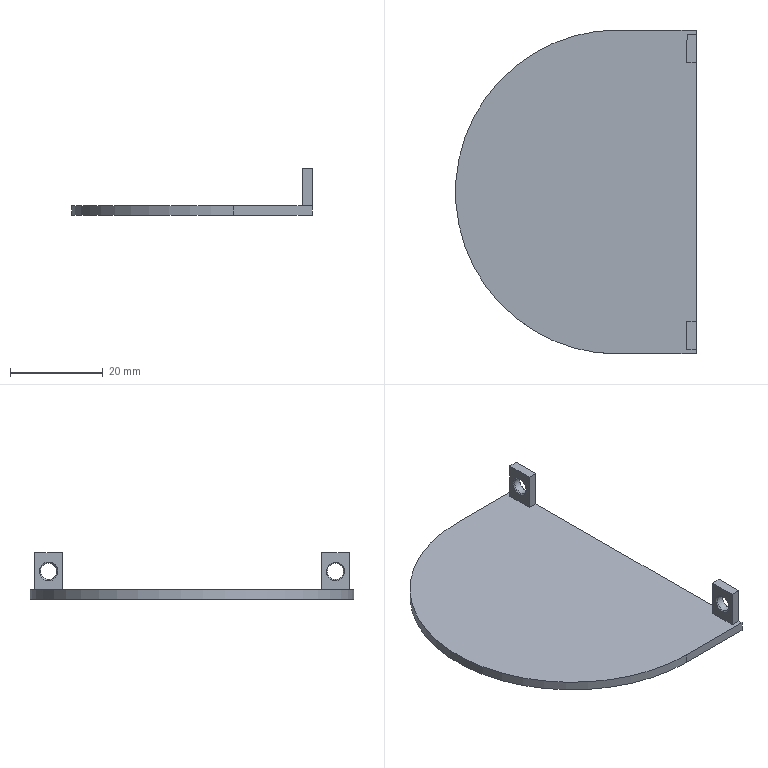Component | NX | LOCK_BODY_BASE_COVER | 1 solid | 20 faces | volume 6380 mm3 | plane 13 | cone 4 | cylinder 3 | commonest cylinder face diameters 3.5 x2 70 x1